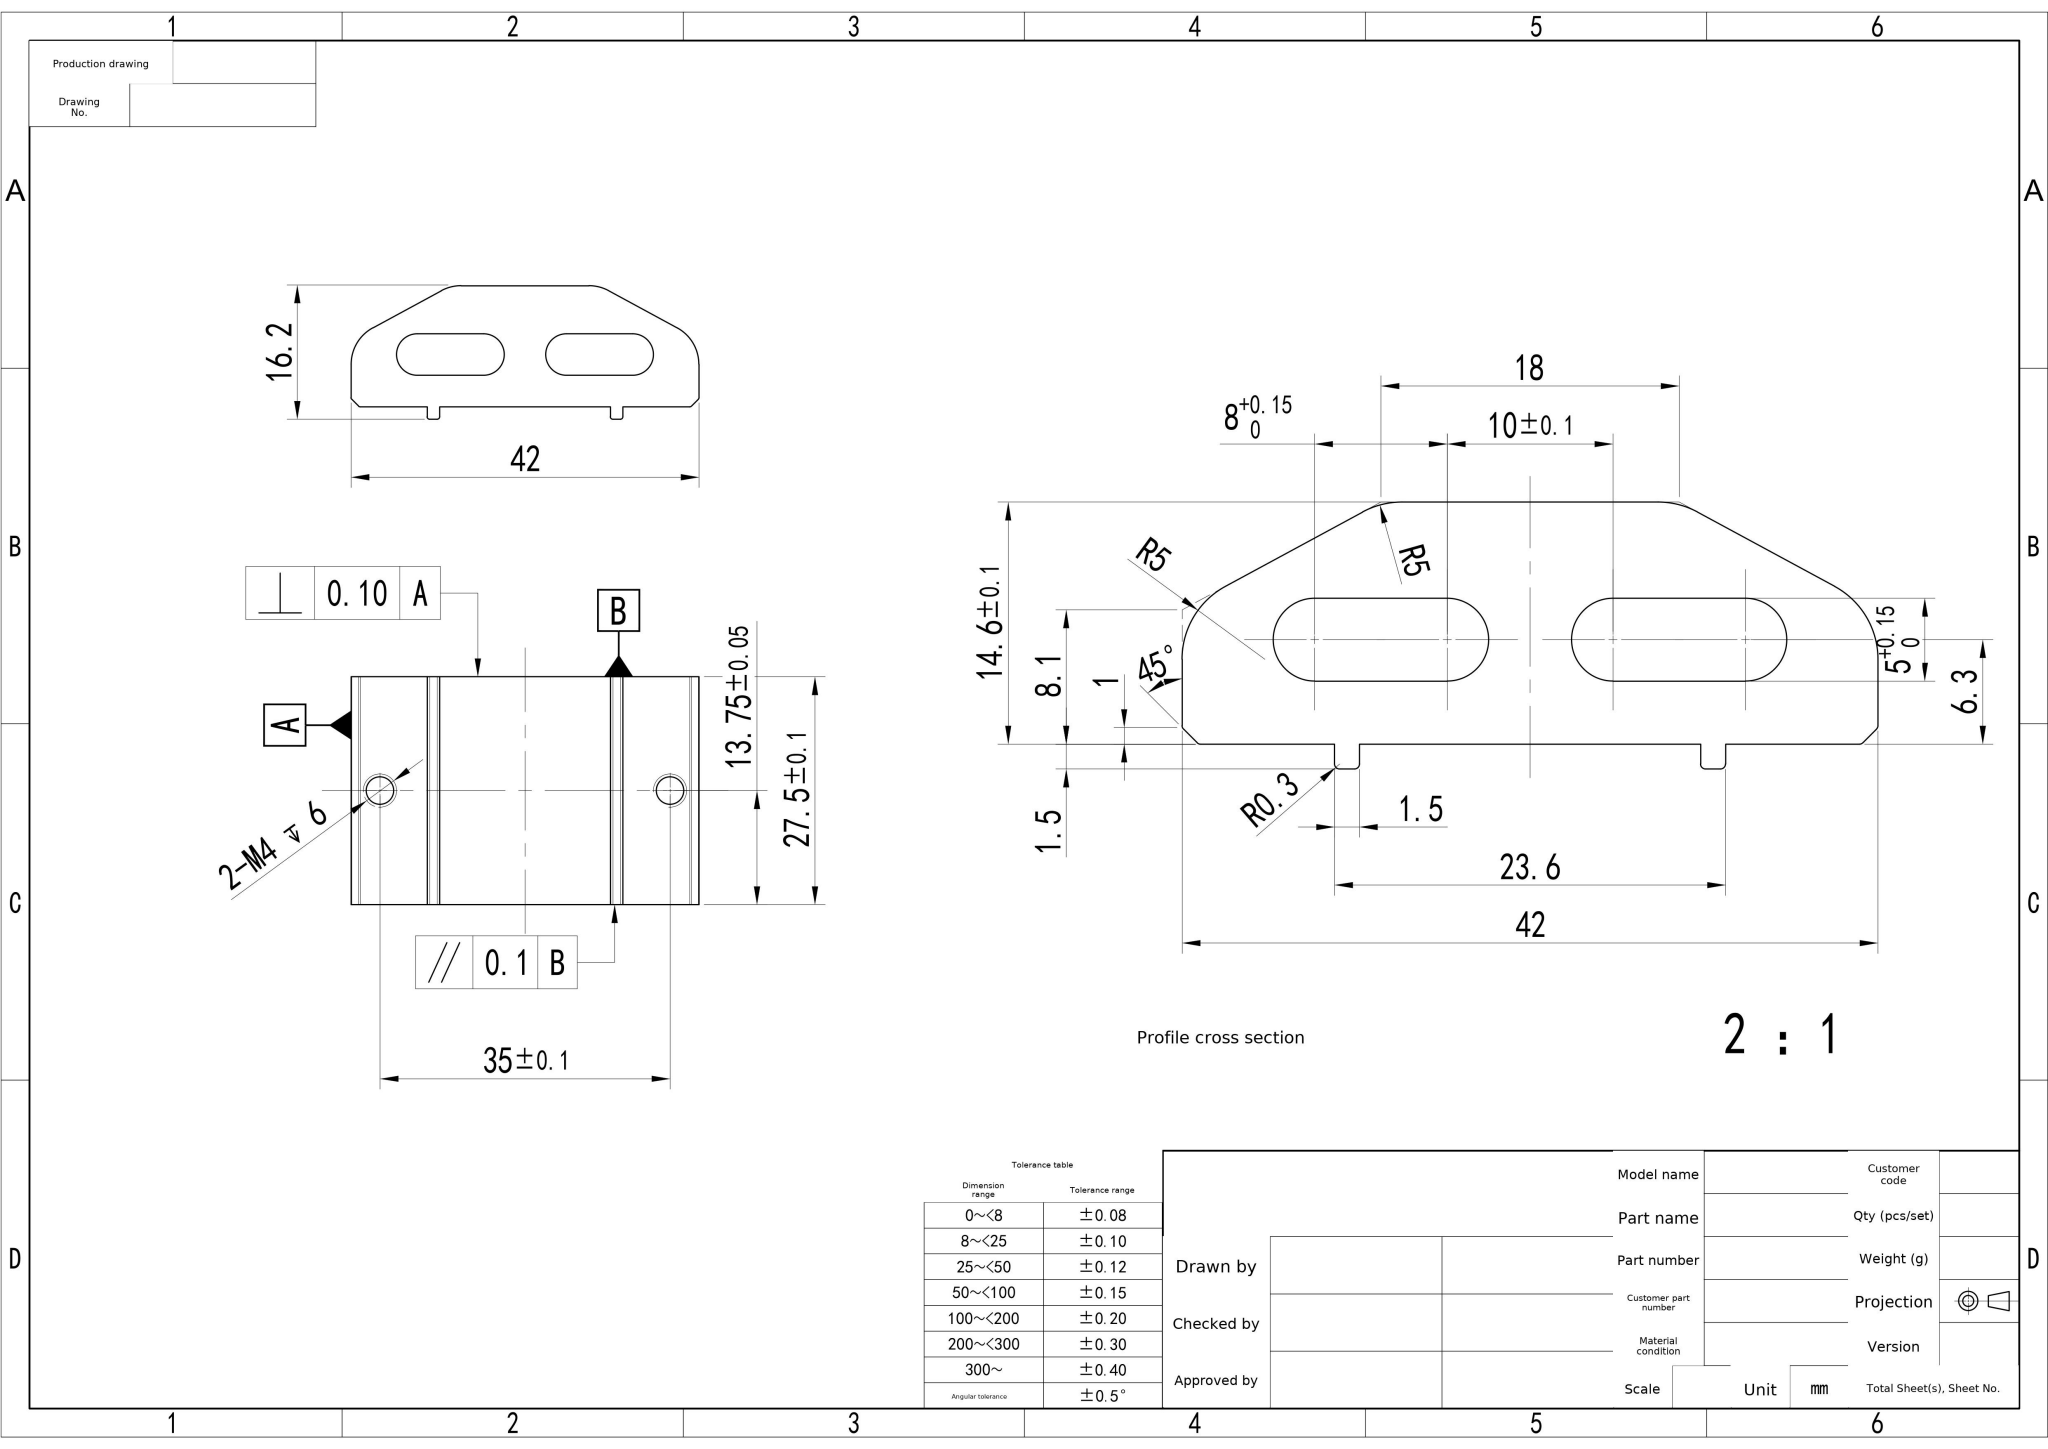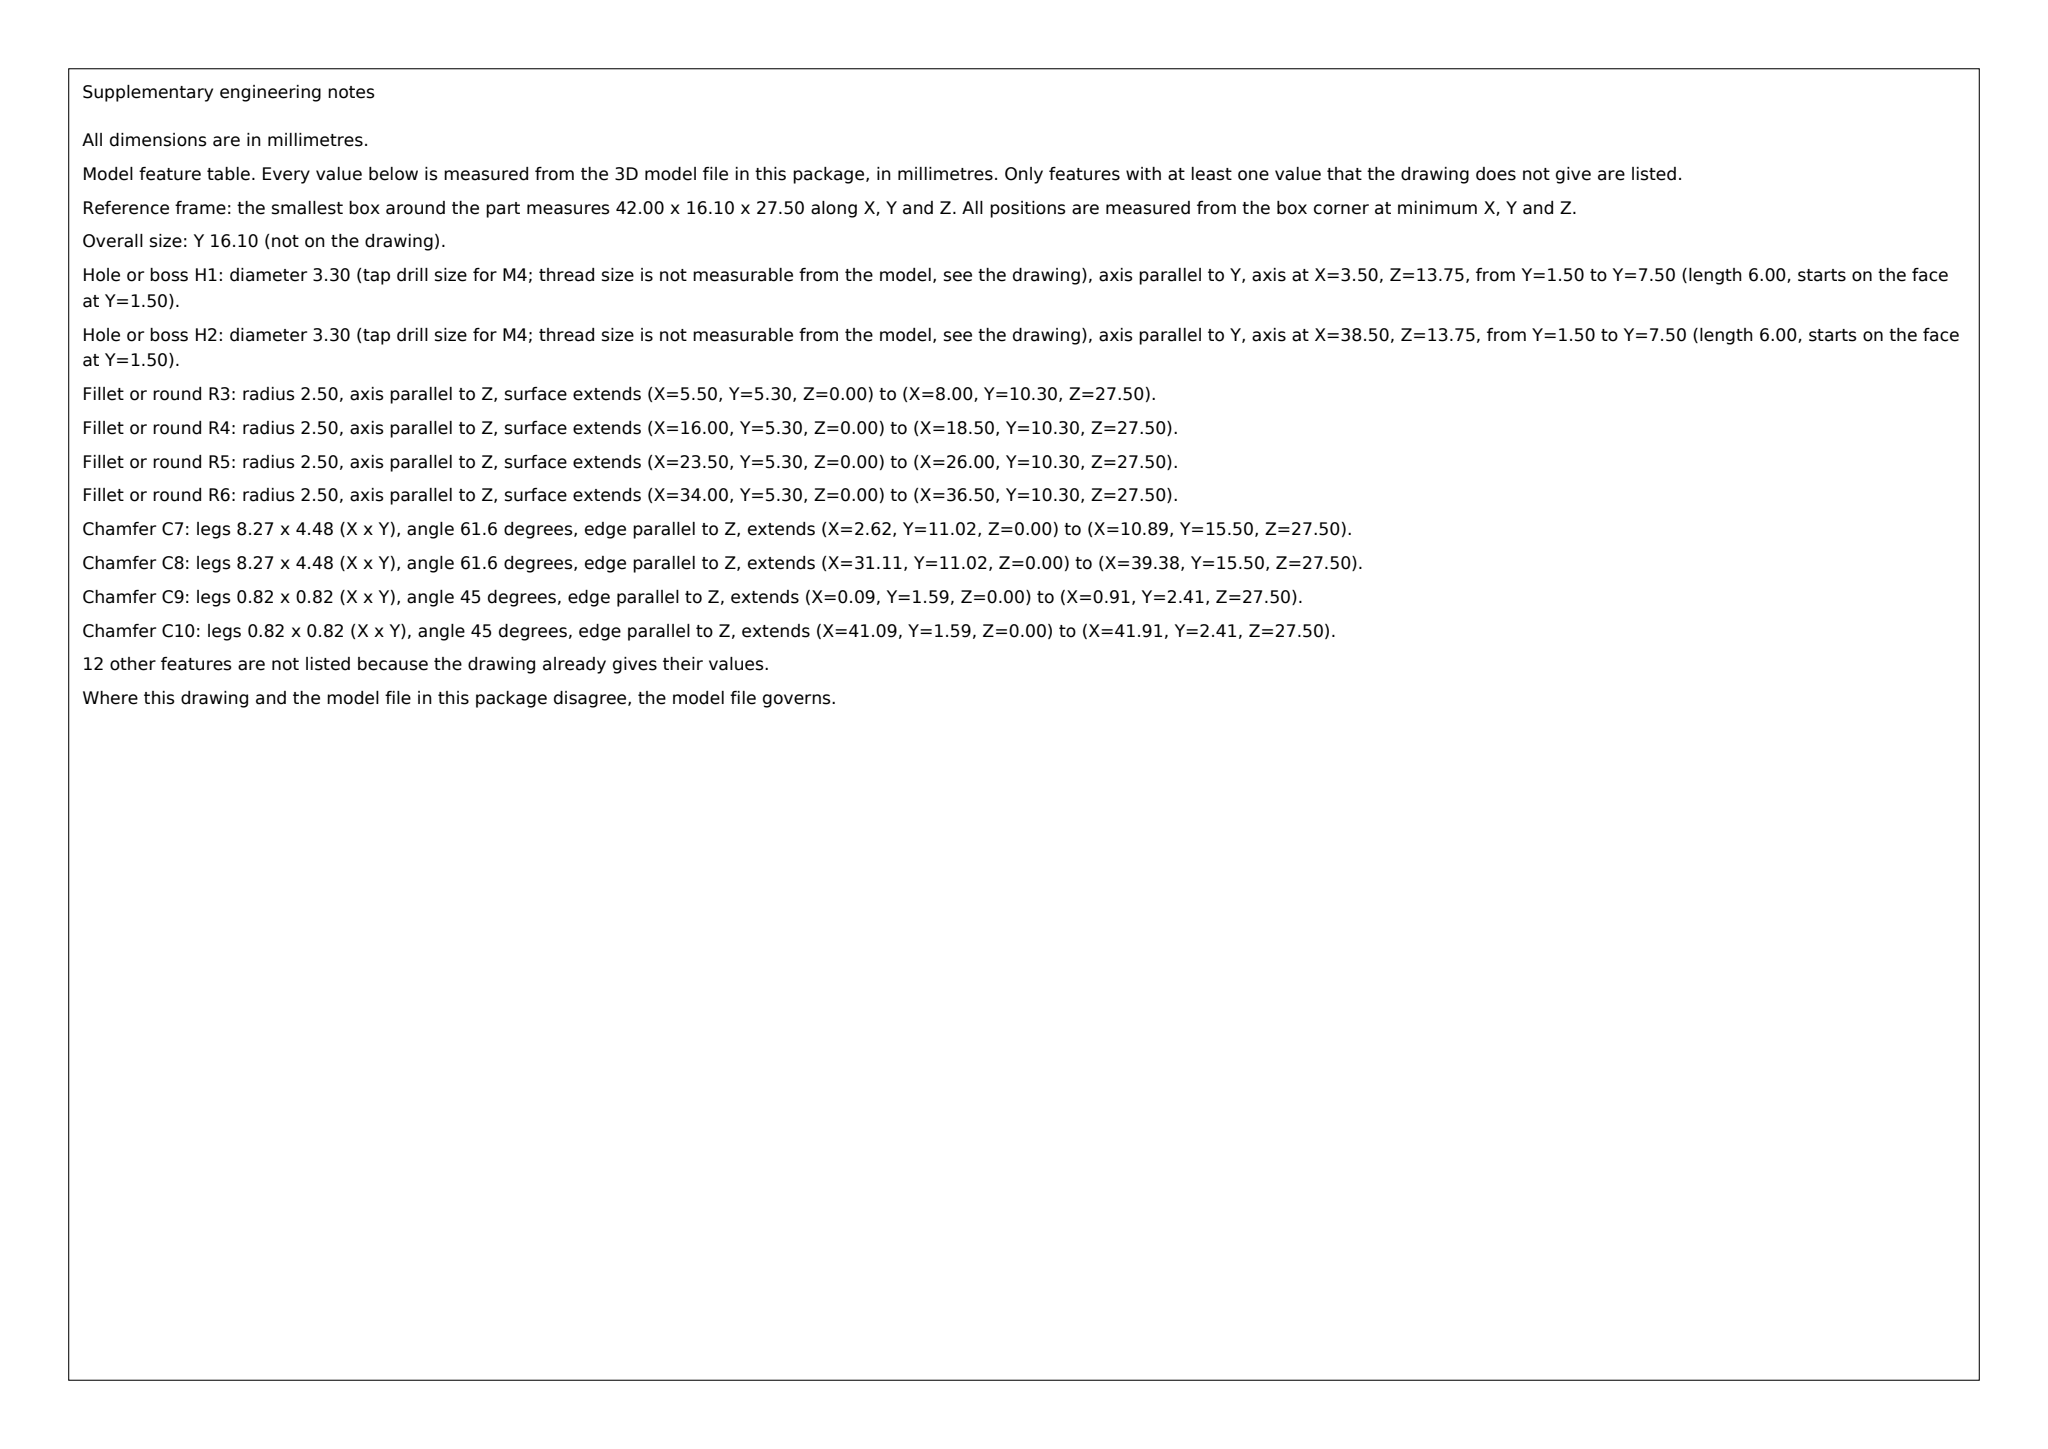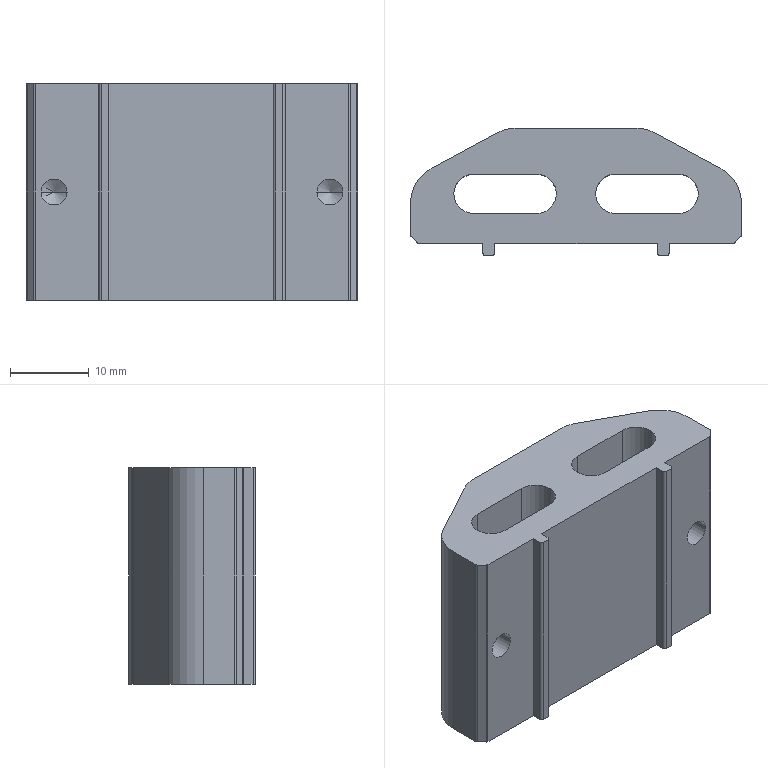Part | SolidWorks | mm | 1 solid | 48 faces | box 42 x 16.1 x 27.5 mm | volume 11336 mm3 | cylinder 22 | plane 22 | cone 4 | commonest cylinder face diameters 0.6 x8 5 x6 3.3 x4 10 x4